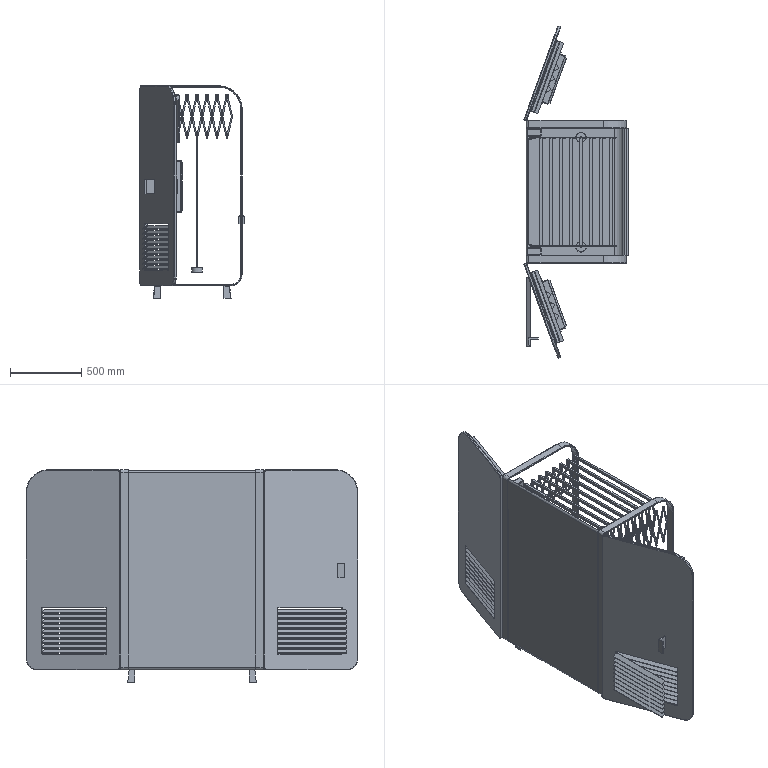Assembly | NX | mm | 39 component files | 163 solids | 1745 faces | box 728.54 x 2321.48 x 1486 mm | volume 72134515 mm3 | plane 1111 | cylinder 580 | torus 54 | commonest cylinder face diameters 4 x209 6 x124 10 x108 18 x54 8 x16 200 x16 40 x10 9 x8
Bill of materials:
unnamed part 1 | 2 |  | Flanged cap/plug shape: thin square plate with rounded corners on top, a slightly smaller thin step under it, and a cylindrical body below with a rounded bottom edge.
unnamed part 2 | 1 |  | Long straight prismatic bar with a constant cross-section: rounded top corners, flat sides and bottom, and a narrow slot running up from the bottom to about mid-height along the whole length.
unnamed part 3 | 1 |  | Very thin flat rectangular plate or sheet with no visible holes or features.
unnamed part 4 | 1 |  | Dumbbell-like part: a thin straight cylindrical rod with a short, larger-diameter cylindrical disc at each end.
unnamed part 5 | 2 |  | Prismatic block with a rectangular notch or step cut into one side, two chamfered corners on one end, and a short cylindrical boss sticking out from the notched face.
unnamed part 6 | 8 |  | Long slender square-section bar with a row of evenly spaced small circular holes along one face and a small pin-like stub at each end.
unnamed part 7 | 1 |  | Thin rectangular plate or panel with one large-radius rounded corner and small edge radii, with a louvered grille of about 10 parallel slots near one end.
unnamed part 8 | 2 |  | Set of 17 separate small identical cylindrical pins, arranged in two parallel staggered rows of 9 and 8.
unnamed part 9 | 1 |  | Thin-walled open-ended tubular shell or sleeve. Its rectangular cross-section has one large-radius rounded corner and small radii at the other corners.
unnamed part 10 | 1 |  | Scissor (lazy-tongs) style lattice of flat straight bars crossing in a repeating X/diamond pattern, with small holes at the bar ends and crossing points.
unnamed part 11 | 2 |  | Solid rectangular block with chamfered edges along some edges, mostly at one end and along the top and bottom long edges.
unnamed part 12 | 2 |  | Long slender straight channel extrusion with a C/U-shaped cross-section.
unnamed part 13 | 2 |  | Very thin flat circular disc, drawn as a faceted polygon with about 20 sides.
unnamed part 14 | 2 |  | Flat rectangular panel with a stepped rail running along its top edge. The rail has a rounded bead/hook profile. The face has a grid of shallow score lines or grooves.
unnamed part 15 | 1 |  | Several separate bodies spread out in space: a scissor-type crossed-link lattice, a set of parallel thin slats, and several small block- and plate-like pieces.
unnamed part 16 | 2 |  | Two separate L-section angle pieces of similar size. One has a notch or step cut into one flange.
unnamed part 17 | 2 |  | Thick rectangular block/plate with chamfered edges. The top face has three small square recesses. The large front face has a circular pattern of radial slits/segments, like a fan or iris.
unnamed part 18 | 4 |  | Solid square frustum: a tapered square prism whose top face is smaller than its base.
unnamed part 19 | 1 |  | Thin rectangular plate with one large rounded corner. It has an array of about 10 parallel slots near one end and a slightly raised or stepped region on one face.
unnamed part 20 | 1 |  | Flat scissor (lazy-tongs) lattice of straight crossed links, with small pivot holes at the link ends and crossing points. It forms a row of about 8 to 9 diamond cells.
Mates:
1. fix | assembly component
2. bond | cross_bar 8 component | assembly component
3. bond | cross_bar 7 component | assembly component
4. linear | assembly datumaxis | assembly cartesiancoordinatesystem | assembly cartesiancoordinatesystem | assembly cartesiancoordinatesystem | assembly cartesiancoordinatesystem | assembly cartesiancoordinatesystem | assembly cartesiancoordinatesystem | assembly cartesiancoordinatesystem | assembly cartesiancoordinatesystem
5. bond | cross_bar 6 component | assembly component
6. bond | cross_bar 5 component | assembly component
7. bond | cross_bar 4 component | assembly component
8. bond | cross_bar 3 component | assembly component
9. bond | cross_bar 2 component | assembly component
10. bond | cross_bar 1 component | assembly component